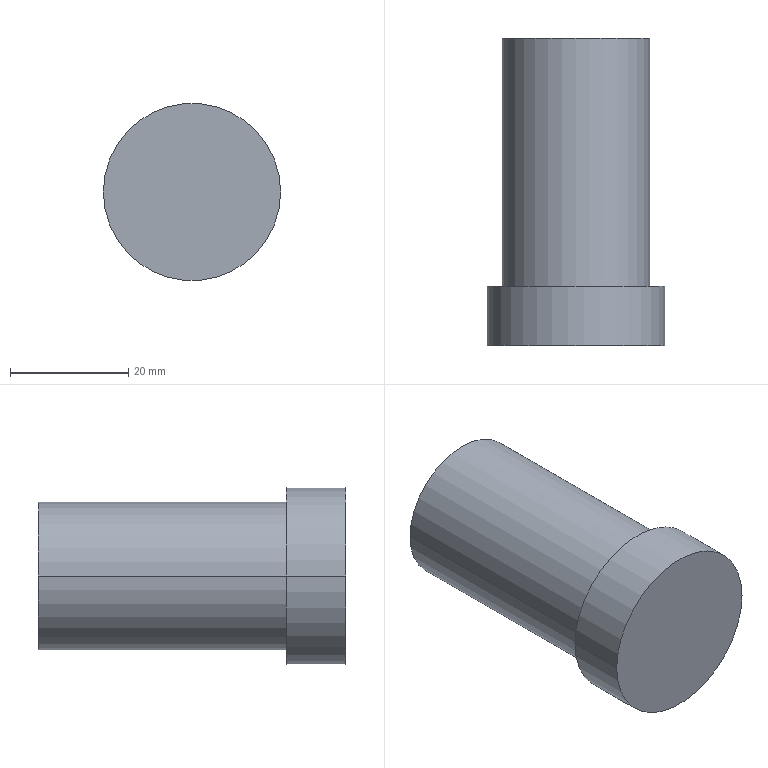Component | SolidWorks | FlipAxisOne-4 | 1 solid | 7 faces | box 30 x 52 x 30 mm | volume 27685 mm3 | cylinder 4 | plane 3 | commonest cylinder face diameters 25 x2 30 x2 | material Plain Carbon Steel
build123d program:
from build123d import *

# Parameters (mm, degrees)
SKETCH1_R           = 15
BOSS_EXTRUDE1_DEPTH = 10
SKETCH2_R           = 12.5
BOSS_EXTRUDE2_DEPTH = 42


with BuildPart() as part:
    # Sketch1 → Boss-Extrude1 (new body)
    with BuildSketch(Plane.XY):
        Circle(SKETCH1_R)
    extrude(amount=BOSS_EXTRUDE1_DEPTH)

    # Sketch2 → Boss-Extrude2 (add)
    with BuildSketch(Plane.XY.offset(10)):
        with Locations(Location((0, 0, 0), (0, 0, 180))):
            Circle(SKETCH2_R)
    extrude(amount=BOSS_EXTRUDE2_DEPTH)


solid = part.part

# Placed as in the assembly
solid = solid.moved(Location((-864.885, 542.093, 1035.102), (-90, 0, 0)))
STEP:
#1=COLOUR_RGB('',0.7922,0.8196,0.9333);
#2=FILL_AREA_STYLE_COLOUR('',#1);
#3=FILL_AREA_STYLE('',(#2));
#4=SURFACE_STYLE_FILL_AREA(#3);
#5=SURFACE_SIDE_STYLE('',(#4));
#6=SURFACE_STYLE_USAGE(.BOTH.,#5);
#7=PRESENTATION_STYLE_ASSIGNMENT((#6));
#8=CARTESIAN_POINT('',(-33.558,23.389,40.752));
#9=VERTEX_POINT('',#8);
#10=CARTESIAN_POINT('',(-34.543,23.389,40.752));
#11=VERTEX_POINT('',#10);
#12=CARTESIAN_POINT('',(-34.051,23.389,40.752));
#13=DIRECTION('',(0.,1.,0.));
#14=DIRECTION('',(1.,0.,0.));
#15=AXIS2_PLACEMENT_3D('',#12,#13,#14);
#16=CIRCLE('',#15,0.4921);
#17=EDGE_CURVE('',#9,#11,#16,.T.);
#18=ORIENTED_EDGE('',*,*,#17,.F.);
#19=CARTESIAN_POINT('',(-33.558,21.736,40.752));
#20=VERTEX_POINT('',#19);
#21=CARTESIAN_POINT('',(-33.558,23.389,40.752));
#22=DIRECTION('',(0.,-1.,0.));
#23=VECTOR('',#22,39.37);
#24=LINE('',#21,#23);
#25=EDGE_CURVE('',#9,#20,#24,.T.);
#26=ORIENTED_EDGE('',*,*,#25,.T.);
#27=CARTESIAN_POINT('',(-34.543,21.736,40.752));
#28=VERTEX_POINT('',#27);
#29=CARTESIAN_POINT('',(-34.051,21.736,40.752));
#30=DIRECTION('',(0.,1.,0.));
#31=DIRECTION('',(1.,0.,0.));
#32=AXIS2_PLACEMENT_3D('',#29,#30,#31);
#33=CIRCLE('',#32,0.4921);
#34=EDGE_CURVE('',#20,#28,#33,.T.);
#35=ORIENTED_EDGE('',*,*,#34,.T.);
#36=CARTESIAN_POINT('',(-34.543,23.389,40.752));
#37=DIRECTION('',(0.,-1.,0.));
#38=VECTOR('',#37,39.37);
#39=LINE('',#36,#38);
#40=EDGE_CURVE('',#11,#28,#39,.T.);
#41=ORIENTED_EDGE('',*,*,#40,.F.);
#42=EDGE_LOOP('',(#18,#26,#35,#41));
#43=FACE_OUTER_BOUND('',#42,.T.);
#44=CARTESIAN_POINT('',(-34.051,23.389,40.752));
#45=DIRECTION('',(0.,-1.,0.));
#46=DIRECTION('',(-1.,0.,0.));
#47=AXIS2_PLACEMENT_3D('',#44,#45,#46);
#48=CYLINDRICAL_SURFACE('',#47,0.4921);
#49=ADVANCED_FACE('',(#43),#48,.T.);
#50=CARTESIAN_POINT('',(-33.46,21.736,40.752));
#51=VERTEX_POINT('',#50);
#52=CARTESIAN_POINT('',(-34.641,21.736,40.752));
#53=VERTEX_POINT('',#52);
#54=CARTESIAN_POINT('',(-34.051,21.736,40.752));
#55=DIRECTION('',(0.,1.,0.));
#56=DIRECTION('',(1.,0.,0.));
#57=AXIS2_PLACEMENT_3D('',#54,#55,#56);
#58=CIRCLE('',#57,0.5906);
#59=EDGE_CURVE('',#51,#53,#58,.T.);
#60=ORIENTED_EDGE('',*,*,#59,.F.);
#61=CARTESIAN_POINT('',(-33.46,21.342,40.752));
#62=VERTEX_POINT('',#61);
#63=CARTESIAN_POINT('',(-33.46,21.736,40.752));
#64=DIRECTION('',(0.,-1.,0.));
#65=VECTOR('',#64,39.37);
#66=LINE('',#63,#65);
#67=EDGE_CURVE('',#51,#62,#66,.T.);
#68=ORIENTED_EDGE('',*,*,#67,.T.);
#69=CARTESIAN_POINT('',(-34.641,21.342,40.752));
#70=VERTEX_POINT('',#69);
#71=CARTESIAN_POINT('',(-34.051,21.342,40.752));
#72=DIRECTION('',(0.,1.,0.));
#73=DIRECTION('',(1.,0.,0.));
#74=AXIS2_PLACEMENT_3D('',#71,#72,#73);
#75=CIRCLE('',#74,0.5906);
#76=EDGE_CURVE('',#62,#70,#75,.T.);
#77=ORIENTED_EDGE('',*,*,#76,.T.);
#78=CARTESIAN_POINT('',(-34.641,21.736,40.752));
#79=DIRECTION('',(0.,-1.,0.));
#80=VECTOR('',#79,39.37);
#81=LINE('',#78,#80);
#82=EDGE_CURVE('',#53,#70,#81,.T.);
#83=ORIENTED_EDGE('',*,*,#82,.F.);
#84=EDGE_LOOP('',(#60,#68,#77,#83));
#85=FACE_OUTER_BOUND('',#84,.T.);
#86=CARTESIAN_POINT('',(-34.051,21.736,40.752));
#87=DIRECTION('',(0.,-1.,0.));
#88=DIRECTION('',(-1.,0.,0.));
#89=AXIS2_PLACEMENT_3D('',#86,#87,#88);
#90=CYLINDRICAL_SURFACE('',#89,0.5906);
#91=ADVANCED_FACE('',(#85),#90,.T.);
#92=CARTESIAN_POINT('',(-34.051,21.736,40.752));
#93=DIRECTION('',(0.,1.,0.));
#94=DIRECTION('',(1.,0.,0.));
#95=AXIS2_PLACEMENT_3D('',#92,#93,#94);
#96=CIRCLE('',#95,0.5906);
#97=EDGE_CURVE('',#53,#51,#96,.T.);
#98=ORIENTED_EDGE('',*,*,#97,.T.);
#99=ORIENTED_EDGE('',*,*,#59,.T.);
#100=EDGE_LOOP('',(#98,#99));
#101=FACE_OUTER_BOUND('',#100,.T.);
#102=CARTESIAN_POINT('',(-34.051,21.736,40.752));
#103=DIRECTION('',(0.,1.,0.));
#104=DIRECTION('',(1.,0.,0.));
#105=AXIS2_PLACEMENT_3D('',#102,#103,#104);
#106=CIRCLE('',#105,0.4921);
#107=EDGE_CURVE('',#28,#20,#106,.T.);
#108=ORIENTED_EDGE('',*,*,#107,.F.);
#109=ORIENTED_EDGE('',*,*,#34,.F.);
#110=EDGE_LOOP('',(#108,#109));
#111=FACE_BOUND('',#110,.T.);
#112=CARTESIAN_POINT('',(-34.051,21.736,40.752));
#113=DIRECTION('',(0.,1.,0.));
#114=DIRECTION('',(1.,0.,0.));
#115=AXIS2_PLACEMENT_3D('',#112,#113,#114);
#116=PLANE('',#115);
#117=ADVANCED_FACE('',(#101,#111),#116,.T.);
#118=ORIENTED_EDGE('',*,*,#67,.F.);
#119=ORIENTED_EDGE('',*,*,#97,.F.);
#120=ORIENTED_EDGE('',*,*,#82,.T.);
#121=CARTESIAN_POINT('',(-34.051,21.342,40.752));
#122=DIRECTION('',(0.,1.,0.));
#123=DIRECTION('',(1.,0.,0.));
#124=AXIS2_PLACEMENT_3D('',#121,#122,#123);
#125=CIRCLE('',#124,0.5906);
#126=EDGE_CURVE('',#70,#62,#125,.T.);
#127=ORIENTED_EDGE('',*,*,#126,.T.);
#128=EDGE_LOOP('',(#118,#119,#120,#127));
#129=FACE_OUTER_BOUND('',#128,.T.);
#130=CARTESIAN_POINT('',(-34.051,21.736,40.752));
#131=DIRECTION('',(0.,-1.,0.));
#132=DIRECTION('',(-1.,0.,0.));
#133=AXIS2_PLACEMENT_3D('',#130,#131,#132);
#134=CYLINDRICAL_SURFACE('',#133,0.5906);
#135=ADVANCED_FACE('',(#129),#134,.T.);
#136=ORIENTED_EDGE('',*,*,#126,.F.);
#137=ORIENTED_EDGE('',*,*,#76,.F.);
#138=EDGE_LOOP('',(#136,#137));
#139=FACE_OUTER_BOUND('',#138,.T.);
#140=CARTESIAN_POINT('',(-34.051,21.342,40.752));
#141=DIRECTION('',(0.,1.,0.));
#142=DIRECTION('',(1.,0.,0.));
#143=AXIS2_PLACEMENT_3D('',#140,#141,#142);
#144=PLANE('',#143);
#145=ADVANCED_FACE('',(#139),#144,.F.);
#146=ORIENTED_EDGE('',*,*,#25,.F.);
#147=CARTESIAN_POINT('',(-34.051,23.389,40.752));
#148=DIRECTION('',(0.,1.,0.));
#149=DIRECTION('',(1.,0.,0.));
#150=AXIS2_PLACEMENT_3D('',#147,#148,#149);
#151=CIRCLE('',#150,0.4921);
#152=EDGE_CURVE('',#11,#9,#151,.T.);
#153=ORIENTED_EDGE('',*,*,#152,.F.);
#154=ORIENTED_EDGE('',*,*,#40,.T.);
#155=ORIENTED_EDGE('',*,*,#107,.T.);
#156=EDGE_LOOP('',(#146,#153,#154,#155));
#157=FACE_OUTER_BOUND('',#156,.T.);
#158=CARTESIAN_POINT('',(-34.051,23.389,40.752));
#159=DIRECTION('',(0.,-1.,0.));
#160=DIRECTION('',(-1.,0.,0.));
#161=AXIS2_PLACEMENT_3D('',#158,#159,#160);
#162=CYLINDRICAL_SURFACE('',#161,0.4921);
#163=ADVANCED_FACE('',(#157),#162,.T.);
#164=ORIENTED_EDGE('',*,*,#152,.T.);
#165=ORIENTED_EDGE('',*,*,#17,.T.);
#166=EDGE_LOOP('',(#164,#165));
#167=FACE_OUTER_BOUND('',#166,.T.);
#168=CARTESIAN_POINT('',(-34.051,23.389,40.752));
#169=DIRECTION('',(0.,1.,0.));
#170=DIRECTION('',(1.,0.,0.));
#171=AXIS2_PLACEMENT_3D('',#168,#169,#170);
#172=PLANE('',#171);
#173=ADVANCED_FACE('',(#167),#172,.T.);
#174=CLOSED_SHELL('',(#49,#91,#117,#135,#145,#163,#173));
#175=MANIFOLD_SOLID_BREP('',#174);
#176=STYLED_ITEM('',(#7),#175);
#177=PRESENTATION_LAYER_ASSIGNMENT('','',(#176));
#178=(LENGTH_UNIT()NAMED_UNIT(*)SI_UNIT($,.METRE.));
#179=LENGTH_MEASURE_WITH_UNIT(LENGTH_MEASURE(0.0254),#178);
#180=DIMENSIONAL_EXPONENTS(1.,0.,0.,0.,0.,0.,0.);
#181=(CONVERSION_BASED_UNIT('',#179)LENGTH_UNIT()NAMED_UNIT(#180));
#182=UNCERTAINTY_MEASURE_WITH_UNIT(LENGTH_MEASURE(0.00001),#181,'','');
#183=(NAMED_UNIT(*)PLANE_ANGLE_UNIT()SI_UNIT($,.RADIAN.));
#184=(NAMED_UNIT(*)SI_UNIT($,.STERADIAN.)SOLID_ANGLE_UNIT());
#185=(GEOMETRIC_REPRESENTATION_CONTEXT(3)GLOBAL_UNCERTAINTY_ASSIGNED_CONTEXT((#182))GLOBAL_UNIT_ASSIGNED_CONTEXT((#181,#183,#184))REPRESENTATION_CONTEXT('',''));
#186=MECHANICAL_DESIGN_GEOMETRIC_PRESENTATION_REPRESENTATION('',(#176),#185);
#187=CARTESIAN_POINT('',(0.,0.,0.));
#188=DIRECTION('',(0.,0.,1.));
#189=DIRECTION('',(1.,0.,0.));
#190=AXIS2_PLACEMENT_3D('',#187,#188,#189);
#191=(LENGTH_UNIT()NAMED_UNIT(*)SI_UNIT($,.METRE.));
#192=LENGTH_MEASURE_WITH_UNIT(LENGTH_MEASURE(0.0254),#191);
#193=DIMENSIONAL_EXPONENTS(1.,0.,0.,0.,0.,0.,0.);
#194=(CONVERSION_BASED_UNIT('',#192)LENGTH_UNIT()NAMED_UNIT(#193));
#195=UNCERTAINTY_MEASURE_WITH_UNIT(LENGTH_MEASURE(0.00001),#194,'','');
#196=(NAMED_UNIT(*)PLANE_ANGLE_UNIT()SI_UNIT($,.RADIAN.));
#197=(NAMED_UNIT(*)SI_UNIT($,.STERADIAN.)SOLID_ANGLE_UNIT());
#198=(GEOMETRIC_REPRESENTATION_CONTEXT(3)GLOBAL_UNCERTAINTY_ASSIGNED_CONTEXT((#195))GLOBAL_UNIT_ASSIGNED_CONTEXT((#194,#196,#197))REPRESENTATION_CONTEXT('',''));
#199=ADVANCED_BREP_SHAPE_REPRESENTATION('',(#175,#190),#198);